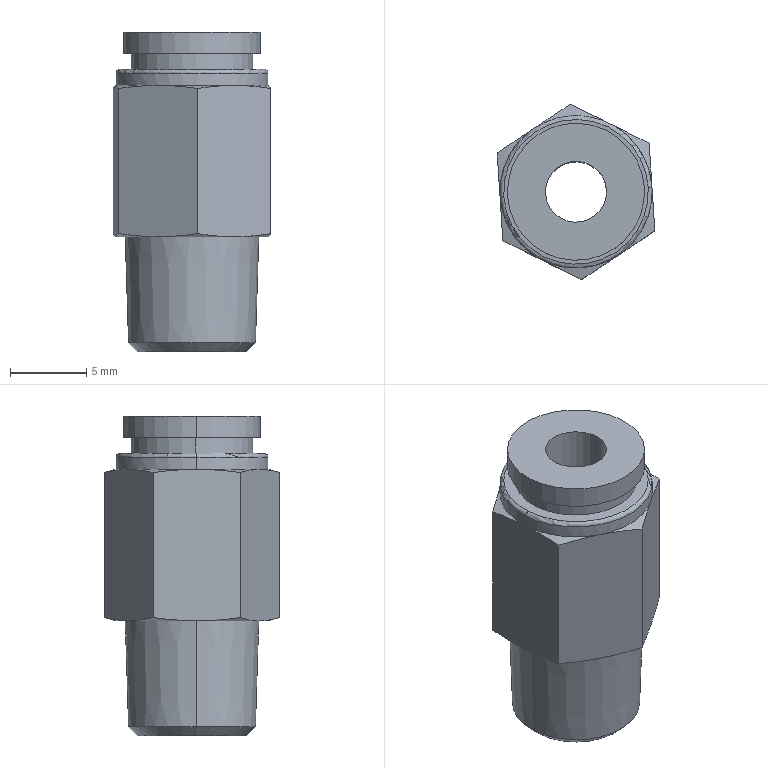Component | SolidWorks | A4-MLCNLSS4-1-L-1 | 1 solid | 37 faces | box 10.35 x 11.52 x 21 mm | volume 1250 mm3 | cone 16 | plane 11 | cylinder 8 | torus 2 | commonest cylinder face diameters 4 x2 9 x2 8 x2 10 x2
STEP:
#1=CARTESIAN_POINT('',(0.07858,-0.3099,2.497));
#2=VERTEX_POINT('',#1);
#3=CARTESIAN_POINT('',(-0.07858,-0.32,2.497));
#4=VERTEX_POINT('',#3);
#5=CARTESIAN_POINT('',(0.,-0.315,2.497));
#6=DIRECTION('',(0.,0.,-1.));
#7=DIRECTION('',(-0.9979,-0.0641,0.));
#8=AXIS2_PLACEMENT_3D('',#5,#6,#7);
#9=CIRCLE('',#8,0.07874);
#10=EDGE_CURVE('',#2,#4,#9,.T.);
#11=ORIENTED_EDGE('',*,*,#10,.F.);
#12=CARTESIAN_POINT('',(0.07858,-0.3099,1.671));
#13=VERTEX_POINT('',#12);
#14=CARTESIAN_POINT('',(0.07858,-0.3099,2.497));
#15=DIRECTION('',(0.,0.,-1.));
#16=VECTOR('',#15,39.37);
#17=LINE('',#14,#16);
#18=EDGE_CURVE('',#2,#13,#17,.T.);
#19=ORIENTED_EDGE('',*,*,#18,.T.);
#20=CARTESIAN_POINT('',(-0.07858,-0.32,1.671));
#21=VERTEX_POINT('',#20);
#22=CARTESIAN_POINT('',(0.,-0.315,1.671));
#23=DIRECTION('',(0.,0.,-1.));
#24=DIRECTION('',(-0.9979,-0.0641,0.));
#25=AXIS2_PLACEMENT_3D('',#22,#23,#24);
#26=CIRCLE('',#25,0.07874);
#27=EDGE_CURVE('',#13,#21,#26,.T.);
#28=ORIENTED_EDGE('',*,*,#27,.T.);
#29=CARTESIAN_POINT('',(-0.07858,-0.32,2.497));
#30=DIRECTION('',(0.,0.,-1.));
#31=VECTOR('',#30,39.37);
#32=LINE('',#29,#31);
#33=EDGE_CURVE('',#4,#21,#32,.T.);
#34=ORIENTED_EDGE('',*,*,#33,.F.);
#35=EDGE_LOOP('',(#11,#19,#28,#34));
#36=FACE_OUTER_BOUND('',#35,.T.);
#37=CARTESIAN_POINT('',(0.,-0.315,2.497));
#38=DIRECTION('',(0.,0.,-1.));
#39=DIRECTION('',(-0.9979,-0.0641,0.));
#40=AXIS2_PLACEMENT_3D('',#37,#38,#39);
#41=CYLINDRICAL_SURFACE('',#40,0.07874);
#42=ADVANCED_FACE('',(#36),#41,.F.);
#43=CARTESIAN_POINT('',(-0.1641,-0.3255,1.694));
#44=VERTEX_POINT('',#43);
#45=CARTESIAN_POINT('',(0.1641,-0.3044,1.694));
#46=VERTEX_POINT('',#45);
#47=CARTESIAN_POINT('',(0.,-0.315,1.694));
#48=DIRECTION('',(0.,0.,-1.));
#49=DIRECTION('',(-0.9979,-0.0641,0.));
#50=AXIS2_PLACEMENT_3D('',#47,#48,#49);
#51=CIRCLE('',#50,0.1644);
#52=EDGE_CURVE('',#44,#46,#51,.T.);
#53=ORIENTED_EDGE('',*,*,#52,.F.);
#54=CARTESIAN_POINT('',(-0.1727,-0.3261,1.969));
#55=VERTEX_POINT('',#54);
#56=CARTESIAN_POINT('',(-0.1727,-0.3261,1.969));
#57=DIRECTION('',(-0.03117,-0.002002,0.9995));
#58=VECTOR('',#57,39.37);
#59=LINE('',#56,#58);
#60=EDGE_CURVE('',#44,#55,#59,.T.);
#61=ORIENTED_EDGE('',*,*,#60,.T.);
#62=CARTESIAN_POINT('',(0.1727,-0.3039,1.969));
#63=VERTEX_POINT('',#62);
#64=CARTESIAN_POINT('',(0.,-0.315,1.969));
#65=DIRECTION('',(0.,0.,-1.));
#66=DIRECTION('',(-0.9979,-0.0641,0.));
#67=AXIS2_PLACEMENT_3D('',#64,#65,#66);
#68=CIRCLE('',#67,0.173);
#69=EDGE_CURVE('',#55,#63,#68,.T.);
#70=ORIENTED_EDGE('',*,*,#69,.T.);
#71=CARTESIAN_POINT('',(0.1727,-0.3039,1.969));
#72=DIRECTION('',(0.03117,0.002002,0.9995));
#73=VECTOR('',#72,39.37);
#74=LINE('',#71,#73);
#75=EDGE_CURVE('',#46,#63,#74,.T.);
#76=ORIENTED_EDGE('',*,*,#75,.F.);
#77=EDGE_LOOP('',(#53,#61,#70,#76));
#78=FACE_OUTER_BOUND('',#77,.T.);
#79=CARTESIAN_POINT('',(0.,-0.315,1.969));
#80=DIRECTION('',(0.,-0.,1.));
#81=DIRECTION('',(0.9979,0.0641,0.));
#82=AXIS2_PLACEMENT_3D('',#79,#80,#81);
#83=CONICAL_SURFACE('',#82,0.173,0.03124);
#84=ADVANCED_FACE('',(#78),#83,.T.);
#85=CARTESIAN_POINT('',(-0.1405,-0.324,1.671));
#86=VERTEX_POINT('',#85);
#87=CARTESIAN_POINT('',(0.1405,-0.3059,1.671));
#88=VERTEX_POINT('',#87);
#89=CARTESIAN_POINT('',(0.,-0.315,1.671));
#90=DIRECTION('',(0.,0.,-1.));
#91=DIRECTION('',(-0.9979,-0.0641,0.));
#92=AXIS2_PLACEMENT_3D('',#89,#90,#91);
#93=CIRCLE('',#92,0.1408);
#94=EDGE_CURVE('',#86,#88,#93,.T.);
#95=ORIENTED_EDGE('',*,*,#94,.F.);
#96=CARTESIAN_POINT('',(-0.1641,-0.3255,1.694));
#97=DIRECTION('',(-0.7057,-0.04533,0.7071));
#98=VECTOR('',#97,39.37);
#99=LINE('',#96,#98);
#100=EDGE_CURVE('',#86,#44,#99,.T.);
#101=ORIENTED_EDGE('',*,*,#100,.T.);
#102=ORIENTED_EDGE('',*,*,#52,.T.);
#103=CARTESIAN_POINT('',(0.1641,-0.3044,1.694));
#104=DIRECTION('',(0.7057,0.04533,0.7071));
#105=VECTOR('',#104,39.37);
#106=LINE('',#103,#105);
#107=EDGE_CURVE('',#88,#46,#106,.T.);
#108=ORIENTED_EDGE('',*,*,#107,.F.);
#109=EDGE_LOOP('',(#95,#101,#102,#108));
#110=FACE_OUTER_BOUND('',#109,.T.);
#111=CARTESIAN_POINT('',(0.,-0.315,1.694));
#112=DIRECTION('',(0.,-0.,1.));
#113=DIRECTION('',(0.9979,0.0641,0.));
#114=AXIS2_PLACEMENT_3D('',#111,#112,#113);
#115=CONICAL_SURFACE('',#114,0.1644,0.7854);
#116=ADVANCED_FACE('',(#110),#115,.T.);
#117=CARTESIAN_POINT('',(-0.1768,-0.3263,2.497));
#118=VERTEX_POINT('',#117);
#119=CARTESIAN_POINT('',(0.1768,-0.3036,2.497));
#120=VERTEX_POINT('',#119);
#121=CARTESIAN_POINT('',(0.,-0.315,2.497));
#122=DIRECTION('',(0.,0.,-1.));
#123=DIRECTION('',(-0.9979,-0.0641,0.));
#124=AXIS2_PLACEMENT_3D('',#121,#122,#123);
#125=CIRCLE('',#124,0.1772);
#126=EDGE_CURVE('',#118,#120,#125,.T.);
#127=ORIENTED_EDGE('',*,*,#126,.T.);
#128=CARTESIAN_POINT('',(0.1768,-0.3036,2.442));
#129=VERTEX_POINT('',#128);
#130=CARTESIAN_POINT('',(0.1768,-0.3036,2.497));
#131=DIRECTION('',(0.,0.,-1.));
#132=VECTOR('',#131,39.37);
#133=LINE('',#130,#132);
#134=EDGE_CURVE('',#120,#129,#133,.T.);
#135=ORIENTED_EDGE('',*,*,#134,.T.);
#136=CARTESIAN_POINT('',(-0.1768,-0.3263,2.442));
#137=VERTEX_POINT('',#136);
#138=CARTESIAN_POINT('',(0.,-0.315,2.442));
#139=DIRECTION('',(0.,0.,-1.));
#140=DIRECTION('',(-0.9979,-0.0641,0.));
#141=AXIS2_PLACEMENT_3D('',#138,#139,#140);
#142=CIRCLE('',#141,0.1772);
#143=EDGE_CURVE('',#137,#129,#142,.T.);
#144=ORIENTED_EDGE('',*,*,#143,.F.);
#145=CARTESIAN_POINT('',(-0.1768,-0.3263,2.497));
#146=DIRECTION('',(0.,0.,-1.));
#147=VECTOR('',#146,39.37);
#148=LINE('',#145,#147);
#149=EDGE_CURVE('',#118,#137,#148,.T.);
#150=ORIENTED_EDGE('',*,*,#149,.F.);
#151=EDGE_LOOP('',(#127,#135,#144,#150));
#152=FACE_OUTER_BOUND('',#151,.T.);
#153=CARTESIAN_POINT('',(0.,-0.315,2.497));
#154=DIRECTION('',(0.,0.,-1.));
#155=DIRECTION('',(-0.9979,-0.0641,0.));
#156=AXIS2_PLACEMENT_3D('',#153,#154,#155);
#157=CYLINDRICAL_SURFACE('',#156,0.1772);
#158=ADVANCED_FACE('',(#152),#157,.T.);
#159=CARTESIAN_POINT('',(-0.1572,-0.3251,2.442));
#160=VERTEX_POINT('',#159);
#161=CARTESIAN_POINT('',(0.1572,-0.3049,2.442));
#162=VERTEX_POINT('',#161);
#163=CARTESIAN_POINT('',(0.,-0.315,2.442));
#164=DIRECTION('',(0.,0.,-1.));
#165=DIRECTION('',(-0.9979,-0.0641,0.));
#166=AXIS2_PLACEMENT_3D('',#163,#164,#165);
#167=CIRCLE('',#166,0.1575);
#168=EDGE_CURVE('',#160,#162,#167,.T.);
#169=ORIENTED_EDGE('',*,*,#168,.T.);
#170=CARTESIAN_POINT('',(0.1572,-0.3049,2.401));
#171=VERTEX_POINT('',#170);
#172=CARTESIAN_POINT('',(0.1572,-0.3049,2.497));
#173=DIRECTION('',(0.,0.,-1.));
#174=VECTOR('',#173,39.37);
#175=LINE('',#172,#174);
#176=EDGE_CURVE('',#162,#171,#175,.T.);
#177=ORIENTED_EDGE('',*,*,#176,.T.);
#178=CARTESIAN_POINT('',(-0.1572,-0.3251,2.401));
#179=VERTEX_POINT('',#178);
#180=CARTESIAN_POINT('',(0.,-0.315,2.401));
#181=DIRECTION('',(0.,0.,-1.));
#182=DIRECTION('',(-0.9979,-0.0641,0.));
#183=AXIS2_PLACEMENT_3D('',#180,#181,#182);
#184=CIRCLE('',#183,0.1575);
#185=EDGE_CURVE('',#179,#171,#184,.T.);
#186=ORIENTED_EDGE('',*,*,#185,.F.);
#187=CARTESIAN_POINT('',(-0.1572,-0.3251,2.497));
#188=DIRECTION('',(0.,0.,-1.));
#189=VECTOR('',#188,39.37);
#190=LINE('',#187,#189);
#191=EDGE_CURVE('',#160,#179,#190,.T.);
#192=ORIENTED_EDGE('',*,*,#191,.F.);
#193=EDGE_LOOP('',(#169,#177,#186,#192));
#194=FACE_OUTER_BOUND('',#193,.T.);
#195=CARTESIAN_POINT('',(0.,-0.315,2.497));
#196=DIRECTION('',(0.,0.,-1.));
#197=DIRECTION('',(-0.9979,-0.0641,0.));
#198=AXIS2_PLACEMENT_3D('',#195,#196,#197);
#199=CYLINDRICAL_SURFACE('',#198,0.1575);
#200=ADVANCED_FACE('',(#194),#199,.T.);
#201=CARTESIAN_POINT('',(-0.1866,-0.3269,2.401));
#202=VERTEX_POINT('',#201);
#203=CARTESIAN_POINT('',(0.1866,-0.303,2.401));
#204=VERTEX_POINT('',#203);
#205=CARTESIAN_POINT('',(0.,-0.315,2.401));
#206=DIRECTION('',(0.,0.,-1.));
#207=DIRECTION('',(-0.9979,-0.0641,0.));
#208=AXIS2_PLACEMENT_3D('',#205,#206,#207);
#209=CIRCLE('',#208,0.187);
#210=EDGE_CURVE('',#202,#204,#209,.T.);
#211=ORIENTED_EDGE('',*,*,#210,.T.);
#212=CARTESIAN_POINT('',(0.1964,-0.3023,2.391));
#213=VERTEX_POINT('',#212);
#214=CARTESIAN_POINT('',(0.1866,-0.303,2.391));
#215=DIRECTION('',(-0.0641,0.9979,0.));
#216=DIRECTION('',(-0.9979,-0.0641,0.));
#217=AXIS2_PLACEMENT_3D('',#214,#215,#216);
#218=CIRCLE('',#217,0.009843);
#219=EDGE_CURVE('',#204,#213,#218,.T.);
#220=ORIENTED_EDGE('',*,*,#219,.T.);
#221=CARTESIAN_POINT('',(-0.1964,-0.3276,2.391));
#222=VERTEX_POINT('',#221);
#223=CARTESIAN_POINT('',(0.,-0.315,2.391));
#224=DIRECTION('',(0.,0.,-1.));
#225=DIRECTION('',(-0.9979,-0.0641,0.));
#226=AXIS2_PLACEMENT_3D('',#223,#224,#225);
#227=CIRCLE('',#226,0.1969);
#228=EDGE_CURVE('',#222,#213,#227,.T.);
#229=ORIENTED_EDGE('',*,*,#228,.F.);
#230=CARTESIAN_POINT('',(-0.1866,-0.3269,2.391));
#231=DIRECTION('',(0.0641,-0.9979,-0.));
#232=DIRECTION('',(0.9979,0.0641,0.));
#233=AXIS2_PLACEMENT_3D('',#230,#231,#232);
#234=CIRCLE('',#233,0.009843);
#235=EDGE_CURVE('',#202,#222,#234,.T.);
#236=ORIENTED_EDGE('',*,*,#235,.F.);
#237=EDGE_LOOP('',(#211,#220,#229,#236));
#238=FACE_OUTER_BOUND('',#237,.T.);
#239=CARTESIAN_POINT('',(0.,-0.315,2.391));
#240=DIRECTION('',(0.,0.,-1.));
#241=DIRECTION('',(-0.9979,-0.0641,-0.));
#242=AXIS2_PLACEMENT_3D('',#239,#240,#241);
#243=TOROIDAL_SURFACE('',#242,0.187,0.009843);
#244=ADVANCED_FACE('',(#238),#243,.T.);
#245=ORIENTED_EDGE('',*,*,#228,.T.);
#246=CARTESIAN_POINT('',(0.1964,-0.3023,2.36));
#247=VERTEX_POINT('',#246);
#248=CARTESIAN_POINT('',(0.1964,-0.3023,2.497));
#249=DIRECTION('',(0.,0.,-1.));
#250=VECTOR('',#249,39.37);
#251=LINE('',#248,#250);
#252=EDGE_CURVE('',#213,#247,#251,.T.);
#253=ORIENTED_EDGE('',*,*,#252,.T.);
#254=CARTESIAN_POINT('',(0.08729,-0.1385,2.36));
#255=VERTEX_POINT('',#254);
#256=CARTESIAN_POINT('',(0.,-0.315,2.36));
#257=DIRECTION('',(0.,0.,-1.));
#258=DIRECTION('',(-0.9979,-0.0641,0.));
#259=AXIS2_PLACEMENT_3D('',#256,#257,#258);
#260=CIRCLE('',#259,0.1969);
#261=EDGE_CURVE('',#255,#247,#260,.T.);
#262=ORIENTED_EDGE('',*,*,#261,.F.);
#263=CARTESIAN_POINT('',(-0.1092,-0.1511,2.36));
#264=VERTEX_POINT('',#263);
#265=CARTESIAN_POINT('',(0.,-0.315,2.36));
#266=DIRECTION('',(0.,0.,-1.));
#267=DIRECTION('',(-0.9979,-0.0641,0.));
#268=AXIS2_PLACEMENT_3D('',#265,#266,#267);
#269=CIRCLE('',#268,0.1969);
#270=EDGE_CURVE('',#264,#255,#269,.T.);
#271=ORIENTED_EDGE('',*,*,#270,.F.);
#272=CARTESIAN_POINT('',(-0.1964,-0.3276,2.36));
#273=VERTEX_POINT('',#272);
#274=CARTESIAN_POINT('',(0.,-0.315,2.36));
#275=DIRECTION('',(0.,0.,-1.));
#276=DIRECTION('',(-0.9979,-0.0641,0.));
#277=AXIS2_PLACEMENT_3D('',#274,#275,#276);
#278=CIRCLE('',#277,0.1969);
#279=EDGE_CURVE('',#273,#264,#278,.T.);
#280=ORIENTED_EDGE('',*,*,#279,.F.);
#281=CARTESIAN_POINT('',(-0.1964,-0.3276,2.497));
#282=DIRECTION('',(0.,0.,-1.));
#283=VECTOR('',#282,39.37);
#284=LINE('',#281,#283);
#285=EDGE_CURVE('',#222,#273,#284,.T.);
#286=ORIENTED_EDGE('',*,*,#285,.F.);
#287=EDGE_LOOP('',(#245,#253,#262,#271,#280,#286));
#288=FACE_OUTER_BOUND('',#287,.T.);
#289=CARTESIAN_POINT('',(0.,-0.315,2.497));
#290=DIRECTION('',(0.,0.,-1.));
#291=DIRECTION('',(-0.9979,-0.0641,0.));
#292=AXIS2_PLACEMENT_3D('',#289,#290,#291);
#293=CYLINDRICAL_SURFACE('',#292,0.1969);
#294=ADVANCED_FACE('',(#288),#293,.T.);
#295=ORIENTED_EDGE('',*,*,#126,.F.);
#296=CARTESIAN_POINT('',(0.,-0.315,2.497));
#297=DIRECTION('',(0.,0.,-1.));
#298=DIRECTION('',(-0.9979,-0.0641,0.));
#299=AXIS2_PLACEMENT_3D('',#296,#297,#298);
#300=CIRCLE('',#299,0.1772);
#301=EDGE_CURVE('',#120,#118,#300,.T.);
#302=ORIENTED_EDGE('',*,*,#301,.F.);
#303=EDGE_LOOP('',(#295,#302));
#304=FACE_OUTER_BOUND('',#303,.T.);
#305=CARTESIAN_POINT('',(0.,-0.315,2.497));
#306=DIRECTION('',(0.,0.,-1.));
#307=DIRECTION('',(-0.9979,-0.0641,0.));
#308=AXIS2_PLACEMENT_3D('',#305,#306,#307);
#309=CIRCLE('',#308,0.07874);
#310=EDGE_CURVE('',#4,#2,#309,.T.);
#311=ORIENTED_EDGE('',*,*,#310,.T.);
#312=ORIENTED_EDGE('',*,*,#10,.T.);
#313=EDGE_LOOP('',(#311,#312));
#314=FACE_BOUND('',#313,.T.);
#315=CARTESIAN_POINT('',(-0.01136,-0.1382,2.497));
#316=DIRECTION('',(0.,0.,-1.));
#317=DIRECTION('',(-0.9979,-0.0641,-0.));
#318=AXIS2_PLACEMENT_3D('',#315,#316,#317);
#319=PLANE('',#318);
#320=ADVANCED_FACE('',(#304,#314),#319,.F.);
#321=CARTESIAN_POINT('',(0.,-0.315,1.671));
#322=DIRECTION('',(0.,0.,-1.));
#323=DIRECTION('',(-0.9979,-0.0641,0.));
#324=AXIS2_PLACEMENT_3D('',#321,#322,#323);
#325=CIRCLE('',#324,0.1408);
#326=EDGE_CURVE('',#88,#86,#325,.T.);
#327=ORIENTED_EDGE('',*,*,#326,.T.);
#328=ORIENTED_EDGE('',*,*,#94,.T.);
#329=EDGE_LOOP('',(#327,#328));
#330=FACE_OUTER_BOUND('',#329,.T.);
#331=CARTESIAN_POINT('',(0.,-0.315,1.671));
#332=DIRECTION('',(0.,0.,-1.));
#333=DIRECTION('',(-0.9979,-0.0641,0.));
#334=AXIS2_PLACEMENT_3D('',#331,#332,#333);
#335=CIRCLE('',#334,0.07874);
#336=EDGE_CURVE('',#21,#13,#335,.T.);
#337=ORIENTED_EDGE('',*,*,#336,.F.);
#338=ORIENTED_EDGE('',*,*,#27,.F.);
#339=EDGE_LOOP('',(#337,#338));
#340=FACE_BOUND('',#339,.T.);
#341=CARTESIAN_POINT('',(0.,-0.315,1.671));
#342=DIRECTION('',(-0.,-0.,1.));
#343=DIRECTION('',(0.9979,0.0641,0.));
#344=AXIS2_PLACEMENT_3D('',#341,#342,#343);
#345=PLANE('',#344);
#346=ADVANCED_FACE('',(#330,#340),#345,.F.);
#347=CARTESIAN_POINT('',(-0.2037,-0.2142,2.352));
#348=VERTEX_POINT('',#347);
#349=CARTESIAN_POINT('',(-0.2037,-0.2142,2.352));
#350=CARTESIAN_POINT('',(-0.1722,-0.1932,2.357));
#351=CARTESIAN_POINT('',(-0.1407,-0.1721,2.36));
#352=CARTESIAN_POINT('',(-0.1092,-0.1511,2.36));
#353=B_SPLINE_CURVE_WITH_KNOTS('',3,(#349,#350,#351,#352),.UNSPECIFIED.,.F.,.F.,(4,4),(0.00000023,0.002887),.UNSPECIFIED.);
#354=EDGE_CURVE('',#348,#264,#353,.T.);
#355=ORIENTED_EDGE('',*,*,#354,.F.);
#356=CARTESIAN_POINT('',(-0.1964,-0.3276,2.36));
#357=CARTESIAN_POINT('',(-0.1989,-0.2897,2.36));
#358=CARTESIAN_POINT('',(-0.2013,-0.2519,2.357));
#359=CARTESIAN_POINT('',(-0.2037,-0.2142,2.352));
#360=B_SPLINE_CURVE_WITH_KNOTS('',3,(#356,#357,#358,#359),.UNSPECIFIED.,.F.,.F.,(4,4),(0.007734,0.01065),.UNSPECIFIED.);
#361=EDGE_CURVE('',#273,#348,#360,.T.);
#362=ORIENTED_EDGE('',*,*,#361,.F.);
#363=ORIENTED_EDGE('',*,*,#279,.T.);
#364=EDGE_LOOP('',(#355,#362,#363));
#365=FACE_OUTER_BOUND('',#364,.T.);
#366=CARTESIAN_POINT('',(0.,-0.315,2.36));
#367=DIRECTION('',(0.,0.,-1.));
#368=DIRECTION('',(-0.9979,-0.0641,0.));
#369=AXIS2_PLACEMENT_3D('',#366,#367,#368);
#370=CONICAL_SURFACE('',#369,0.1969,1.309);
#371=ADVANCED_FACE('',(#365),#370,.T.);
#372=CARTESIAN_POINT('',(-0.01457,-0.08812,2.352));
#373=VERTEX_POINT('',#372);
#374=CARTESIAN_POINT('',(-0.1092,-0.1511,2.36));
#375=CARTESIAN_POINT('',(-0.07762,-0.1301,2.36));
#376=CARTESIAN_POINT('',(-0.0461,-0.1091,2.357));
#377=CARTESIAN_POINT('',(-0.01457,-0.08812,2.352));
#378=B_SPLINE_CURVE_WITH_KNOTS('',3,(#374,#375,#376,#377),.UNSPECIFIED.,.F.,.F.,(4,4),(0.002887,0.005774),.UNSPECIFIED.);
#379=EDGE_CURVE('',#264,#373,#378,.T.);
#380=ORIENTED_EDGE('',*,*,#379,.F.);
#381=ORIENTED_EDGE('',*,*,#270,.T.);
#382=CARTESIAN_POINT('',(-0.01457,-0.08812,2.352));
#383=CARTESIAN_POINT('',(0.01938,-0.1049,2.357));
#384=CARTESIAN_POINT('',(0.05334,-0.1217,2.36));
#385=CARTESIAN_POINT('',(0.08729,-0.1385,2.36));
#386=B_SPLINE_CURVE_WITH_KNOTS('',3,(#382,#383,#384,#385),.UNSPECIFIED.,.F.,.F.,(4,4),(0.00000023,0.002887),.UNSPECIFIED.);
#387=EDGE_CURVE('',#373,#255,#386,.T.);
#388=ORIENTED_EDGE('',*,*,#387,.F.);
#389=EDGE_LOOP('',(#380,#381,#388));
#390=FACE_OUTER_BOUND('',#389,.T.);
#391=CARTESIAN_POINT('',(0.,-0.315,2.36));
#392=DIRECTION('',(0.,0.,-1.));
#393=DIRECTION('',(-0.9979,-0.0641,0.));
#394=AXIS2_PLACEMENT_3D('',#391,#392,#393);
#395=CONICAL_SURFACE('',#394,0.1969,1.309);
#396=ADVANCED_FACE('',(#390),#395,.T.);
#397=CARTESIAN_POINT('',(0.1892,-0.1889,2.352));
#398=VERTEX_POINT('',#397);
#399=CARTESIAN_POINT('',(0.08729,-0.1385,2.36));
#400=CARTESIAN_POINT('',(0.1213,-0.1553,2.36));
#401=CARTESIAN_POINT('',(0.1552,-0.1721,2.357));
#402=CARTESIAN_POINT('',(0.1892,-0.1889,2.352));
#403=B_SPLINE_CURVE_WITH_KNOTS('',3,(#399,#400,#401,#402),.UNSPECIFIED.,.F.,.F.,(4,4),(0.002887,0.005774),.UNSPECIFIED.);
#404=EDGE_CURVE('',#255,#398,#403,.T.);
#405=ORIENTED_EDGE('',*,*,#404,.F.);
#406=ORIENTED_EDGE('',*,*,#261,.T.);
#407=CARTESIAN_POINT('',(0.1892,-0.1889,2.352));
#408=CARTESIAN_POINT('',(0.1916,-0.2267,2.357));
#409=CARTESIAN_POINT('',(0.194,-0.2645,2.36));
#410=CARTESIAN_POINT('',(0.1964,-0.3023,2.36));
#411=B_SPLINE_CURVE_WITH_KNOTS('',3,(#407,#408,#409,#410),.UNSPECIFIED.,.F.,.F.,(4,4),(0.01099,0.0139),.UNSPECIFIED.);
#412=EDGE_CURVE('',#398,#247,#411,.T.);
#413=ORIENTED_EDGE('',*,*,#412,.F.);
#414=EDGE_LOOP('',(#405,#406,#413));
#415=FACE_OUTER_BOUND('',#414,.T.);
#416=CARTESIAN_POINT('',(0.,-0.315,2.36));
#417=DIRECTION('',(0.,0.,-1.));
#418=DIRECTION('',(-0.9979,-0.0641,0.));
#419=AXIS2_PLACEMENT_3D('',#416,#417,#418);
#420=CONICAL_SURFACE('',#419,0.1969,1.309);
#421=ADVANCED_FACE('',(#415),#420,.T.);
#422=CARTESIAN_POINT('',(0.2037,-0.4158,2.352));
#423=VERTEX_POINT('',#422);
#424=CARTESIAN_POINT('',(0.1964,-0.3023,2.36));
#425=CARTESIAN_POINT('',(0.1977,-0.3212,2.36));
#426=CARTESIAN_POINT('',(0.1989,-0.3401,2.359));
#427=CARTESIAN_POINT('',(0.2013,-0.378,2.356));
#428=CARTESIAN_POINT('',(0.2025,-0.3969,2.354));
#429=CARTESIAN_POINT('',(0.2037,-0.4158,2.352));
#430=B_SPLINE_CURVE_WITH_KNOTS('',3,(#424,#425,#426,#427,#428,#429),.UNSPECIFIED.,.F.,.F.,(4,2,4),(0.0139,0.01535,0.01679),.UNSPECIFIED.);
#431=EDGE_CURVE('',#247,#423,#430,.T.);
#432=ORIENTED_EDGE('',*,*,#431,.F.);
#433=CARTESIAN_POINT('',(0.1092,-0.4788,2.36));
#434=VERTEX_POINT('',#433);
#435=CARTESIAN_POINT('',(0.,-0.315,2.36));
#436=DIRECTION('',(0.,0.,-1.));
#437=DIRECTION('',(-0.9979,-0.0641,0.));
#438=AXIS2_PLACEMENT_3D('',#435,#436,#437);
#439=CIRCLE('',#438,0.1969);
#440=EDGE_CURVE('',#247,#434,#439,.T.);
#441=ORIENTED_EDGE('',*,*,#440,.T.);
#442=CARTESIAN_POINT('',(0.2037,-0.4158,2.352));
#443=CARTESIAN_POINT('',(0.1722,-0.4368,2.357));
#444=CARTESIAN_POINT('',(0.1407,-0.4578,2.36));
#445=CARTESIAN_POINT('',(0.1092,-0.4788,2.36));
#446=B_SPLINE_CURVE_WITH_KNOTS('',3,(#442,#443,#444,#445),.UNSPECIFIED.,.F.,.F.,(4,4),(0.00000023,0.002887),.UNSPECIFIED.);
#447=EDGE_CURVE('',#423,#434,#446,.T.);
#448=ORIENTED_EDGE('',*,*,#447,.F.);
#449=EDGE_LOOP('',(#432,#441,#448));
#450=FACE_OUTER_BOUND('',#449,.T.);
#451=CARTESIAN_POINT('',(0.,-0.315,2.36));
#452=DIRECTION('',(0.,0.,-1.));
#453=DIRECTION('',(-0.9979,-0.0641,0.));
#454=AXIS2_PLACEMENT_3D('',#451,#452,#453);
#455=CONICAL_SURFACE('',#454,0.1969,1.309);
#456=ADVANCED_FACE('',(#450),#455,.T.);
#457=CARTESIAN_POINT('',(0.01457,-0.5418,2.352));
#458=VERTEX_POINT('',#457);
#459=CARTESIAN_POINT('',(0.1092,-0.4788,2.36));
#460=CARTESIAN_POINT('',(0.07762,-0.4998,2.36));
#461=CARTESIAN_POINT('',(0.0461,-0.5208,2.357));
#462=CARTESIAN_POINT('',(0.01457,-0.5418,2.352));
#463=B_SPLINE_CURVE_WITH_KNOTS('',3,(#459,#460,#461,#462),.UNSPECIFIED.,.F.,.F.,(4,4),(0.002887,0.005774),.UNSPECIFIED.);
#464=EDGE_CURVE('',#434,#458,#463,.T.);
#465=ORIENTED_EDGE('',*,*,#464,.F.);
#466=CARTESIAN_POINT('',(-0.08729,-0.4914,2.36));
#467=VERTEX_POINT('',#466);
#468=CARTESIAN_POINT('',(0.,-0.315,2.36));
#469=DIRECTION('',(0.,0.,-1.));
#470=DIRECTION('',(-0.9979,-0.0641,0.));
#471=AXIS2_PLACEMENT_3D('',#468,#469,#470);
#472=CIRCLE('',#471,0.1969);
#473=EDGE_CURVE('',#434,#467,#472,.T.);
#474=ORIENTED_EDGE('',*,*,#473,.T.);
#475=CARTESIAN_POINT('',(0.01457,-0.5418,2.352));
#476=CARTESIAN_POINT('',(-0.01938,-0.525,2.357));
#477=CARTESIAN_POINT('',(-0.05334,-0.5082,2.36));
#478=CARTESIAN_POINT('',(-0.08729,-0.4914,2.36));
#479=B_SPLINE_CURVE_WITH_KNOTS('',3,(#475,#476,#477,#478),.UNSPECIFIED.,.F.,.F.,(4,4),(0.00000023,0.002887),.UNSPECIFIED.);
#480=EDGE_CURVE('',#458,#467,#479,.T.);
#481=ORIENTED_EDGE('',*,*,#480,.F.);
#482=EDGE_LOOP('',(#465,#474,#481));
#483=FACE_OUTER_BOUND('',#482,.T.);
#484=CARTESIAN_POINT('',(0.,-0.315,2.36));
#485=DIRECTION('',(0.,0.,-1.));
#486=DIRECTION('',(-0.9979,-0.0641,0.));
#487=AXIS2_PLACEMENT_3D('',#484,#485,#486);
#488=CONICAL_SURFACE('',#487,0.1969,1.309);
#489=ADVANCED_FACE('',(#483),#488,.T.);
#490=CARTESIAN_POINT('',(-0.1892,-0.441,2.352));
#491=VERTEX_POINT('',#490);
#492=CARTESIAN_POINT('',(-0.08729,-0.4914,2.36));
#493=CARTESIAN_POINT('',(-0.1213,-0.4746,2.36));
#494=CARTESIAN_POINT('',(-0.1552,-0.4578,2.357));
#495=CARTESIAN_POINT('',(-0.1892,-0.441,2.352));
#496=B_SPLINE_CURVE_WITH_KNOTS('',3,(#492,#493,#494,#495),.UNSPECIFIED.,.F.,.F.,(4,4),(0.002887,0.005774),.UNSPECIFIED.);
#497=EDGE_CURVE('',#467,#491,#496,.T.);
#498=ORIENTED_EDGE('',*,*,#497,.F.);
#499=CARTESIAN_POINT('',(0.,-0.315,2.36));
#500=DIRECTION('',(0.,0.,-1.));
#501=DIRECTION('',(-0.9979,-0.0641,0.));
#502=AXIS2_PLACEMENT_3D('',#499,#500,#501);
#503=CIRCLE('',#502,0.1969);
#504=EDGE_CURVE('',#467,#273,#503,.T.);
#505=ORIENTED_EDGE('',*,*,#504,.T.);
#506=CARTESIAN_POINT('',(-0.1892,-0.441,2.352));
#507=CARTESIAN_POINT('',(-0.1904,-0.4222,2.354));
#508=CARTESIAN_POINT('',(-0.1916,-0.4032,2.356));
#509=CARTESIAN_POINT('',(-0.194,-0.3654,2.359));
#510=CARTESIAN_POINT('',(-0.1952,-0.3465,2.36));
#511=CARTESIAN_POINT('',(-0.1964,-0.3276,2.36));
#512=B_SPLINE_CURVE_WITH_KNOTS('',3,(#506,#507,#508,#509,#510,#511),.UNSPECIFIED.,.F.,.F.,(4,2,4),(0.004834,0.006284,0.007734),.UNSPECIFIED.);
#513=EDGE_CURVE('',#491,#273,#512,.T.);
#514=ORIENTED_EDGE('',*,*,#513,.F.);
#515=EDGE_LOOP('',(#498,#505,#514));
#516=FACE_OUTER_BOUND('',#515,.T.);
#517=CARTESIAN_POINT('',(0.,-0.315,2.36));
#518=DIRECTION('',(0.,0.,-1.));
#519=DIRECTION('',(-0.9979,-0.0641,0.));
#520=AXIS2_PLACEMENT_3D('',#517,#518,#519);
#521=CONICAL_SURFACE('',#520,0.1969,1.309);
#522=ADVANCED_FACE('',(#516),#521,.T.);
#523=ORIENTED_EDGE('',*,*,#252,.F.);
#524=CARTESIAN_POINT('',(0.,-0.315,2.391));
#525=DIRECTION('',(0.,0.,-1.));
#526=DIRECTION('',(-0.9979,-0.0641,0.));
#527=AXIS2_PLACEMENT_3D('',#524,#525,#526);
#528=CIRCLE('',#527,0.1969);
#529=EDGE_CURVE('',#213,#222,#528,.T.);
#530=ORIENTED_EDGE('',*,*,#529,.T.);
#531=ORIENTED_EDGE('',*,*,#285,.T.);
#532=ORIENTED_EDGE('',*,*,#504,.F.);
#533=ORIENTED_EDGE('',*,*,#473,.F.);
#534=ORIENTED_EDGE('',*,*,#440,.F.);
#535=EDGE_LOOP('',(#523,#530,#531,#532,#533,#534));
#536=FACE_OUTER_BOUND('',#535,.T.);
#537=CARTESIAN_POINT('',(0.,-0.315,2.497));
#538=DIRECTION('',(0.,0.,-1.));
#539=DIRECTION('',(-0.9979,-0.0641,0.));
#540=AXIS2_PLACEMENT_3D('',#537,#538,#539);
#541=CYLINDRICAL_SURFACE('',#540,0.1969);
#542=ADVANCED_FACE('',(#536),#541,.T.);
#543=ORIENTED_EDGE('',*,*,#219,.F.);
#544=CARTESIAN_POINT('',(0.,-0.315,2.401));
#545=DIRECTION('',(0.,0.,-1.));
#546=DIRECTION('',(-0.9979,-0.0641,0.));
#547=AXIS2_PLACEMENT_3D('',#544,#545,#546);
#548=CIRCLE('',#547,0.187);
#549=EDGE_CURVE('',#204,#202,#548,.T.);
#550=ORIENTED_EDGE('',*,*,#549,.T.);
#551=ORIENTED_EDGE('',*,*,#235,.T.);
#552=ORIENTED_EDGE('',*,*,#529,.F.);
#553=EDGE_LOOP('',(#543,#550,#551,#552));
#554=FACE_OUTER_BOUND('',#553,.T.);
#555=CARTESIAN_POINT('',(0.,-0.315,2.391));
#556=DIRECTION('',(0.,0.,-1.));
#557=DIRECTION('',(-0.9979,-0.0641,-0.));
#558=AXIS2_PLACEMENT_3D('',#555,#556,#557);
#559=TOROIDAL_SURFACE('',#558,0.187,0.009843);
#560=ADVANCED_FACE('',(#554),#559,.T.);
#561=ORIENTED_EDGE('',*,*,#210,.F.);
#562=ORIENTED_EDGE('',*,*,#549,.F.);
#563=EDGE_LOOP('',(#561,#562));
#564=FACE_OUTER_BOUND('',#563,.T.);
#565=ORIENTED_EDGE('',*,*,#185,.T.);
#566=CARTESIAN_POINT('',(0.,-0.315,2.401));
#567=DIRECTION('',(0.,0.,-1.));
#568=DIRECTION('',(-0.9979,-0.0641,0.));
#569=AXIS2_PLACEMENT_3D('',#566,#567,#568);
#570=CIRCLE('',#569,0.1575);
#571=EDGE_CURVE('',#171,#179,#570,.T.);
#572=ORIENTED_EDGE('',*,*,#571,.T.);
#573=EDGE_LOOP('',(#565,#572));
#574=FACE_BOUND('',#573,.T.);
#575=CARTESIAN_POINT('',(-0.01199,-0.1283,2.401));
#576=DIRECTION('',(0.,0.,-1.));
#577=DIRECTION('',(-0.9979,-0.0641,-0.));
#578=AXIS2_PLACEMENT_3D('',#575,#576,#577);
#579=PLANE('',#578);
#580=ADVANCED_FACE('',(#564,#574),#579,.F.);
#581=ORIENTED_EDGE('',*,*,#176,.F.);
#582=CARTESIAN_POINT('',(0.,-0.315,2.442));
#583=DIRECTION('',(0.,0.,-1.));
#584=DIRECTION('',(-0.9979,-0.0641,0.));
#585=AXIS2_PLACEMENT_3D('',#582,#583,#584);
#586=CIRCLE('',#585,0.1575);
#587=EDGE_CURVE('',#162,#160,#586,.T.);
#588=ORIENTED_EDGE('',*,*,#587,.T.);
#589=ORIENTED_EDGE('',*,*,#191,.T.);
#590=ORIENTED_EDGE('',*,*,#571,.F.);
#591=EDGE_LOOP('',(#581,#588,#589,#590));
#592=FACE_OUTER_BOUND('',#591,.T.);
#593=CARTESIAN_POINT('',(0.,-0.315,2.497));
#594=DIRECTION('',(0.,0.,-1.));
#595=DIRECTION('',(-0.9979,-0.0641,0.));
#596=AXIS2_PLACEMENT_3D('',#593,#594,#595);
#597=CYLINDRICAL_SURFACE('',#596,0.1575);
#598=ADVANCED_FACE('',(#592),#597,.T.);
#599=ORIENTED_EDGE('',*,*,#168,.F.);
#600=ORIENTED_EDGE('',*,*,#587,.F.);
#601=EDGE_LOOP('',(#599,#600));
#602=FACE_BOUND('',#601,.T.);
#603=ORIENTED_EDGE('',*,*,#143,.T.);
#604=CARTESIAN_POINT('',(0.,-0.315,2.442));
#605=DIRECTION('',(0.,0.,-1.));
#606=DIRECTION('',(-0.9979,-0.0641,0.));
#607=AXIS2_PLACEMENT_3D('',#604,#605,#606);
#608=CIRCLE('',#607,0.1772);
#609=EDGE_CURVE('',#129,#137,#608,.T.);
#610=ORIENTED_EDGE('',*,*,#609,.T.);
#611=EDGE_LOOP('',(#603,#610));
#612=FACE_OUTER_BOUND('',#611,.T.);
#613=CARTESIAN_POINT('',(-0.01009,-0.1578,2.442));
#614=DIRECTION('',(-0.,-0.,1.));
#615=DIRECTION('',(0.9979,0.0641,0.));
#616=AXIS2_PLACEMENT_3D('',#613,#614,#615);
#617=PLANE('',#616);
#618=ADVANCED_FACE('',(#602,#612),#617,.F.);
#619=ORIENTED_EDGE('',*,*,#134,.F.);
#620=ORIENTED_EDGE('',*,*,#301,.T.);
#621=ORIENTED_EDGE('',*,*,#149,.T.);
#622=ORIENTED_EDGE('',*,*,#609,.F.);
#623=EDGE_LOOP('',(#619,#620,#621,#622));
#624=FACE_OUTER_BOUND('',#623,.T.);
#625=CARTESIAN_POINT('',(0.,-0.315,2.497));
#626=DIRECTION('',(0.,0.,-1.));
#627=DIRECTION('',(-0.9979,-0.0641,0.));
#628=AXIS2_PLACEMENT_3D('',#625,#626,#627);
#629=CYLINDRICAL_SURFACE('',#628,0.1772);
#630=ADVANCED_FACE('',(#624),#629,.T.);
#631=CARTESIAN_POINT('',(-0.01457,-0.08812,1.977));
#632=VERTEX_POINT('',#631);
#633=CARTESIAN_POINT('',(-0.1092,-0.1511,1.969));
#634=VERTEX_POINT('',#633);
#635=CARTESIAN_POINT('',(-0.01457,-0.08812,1.977));
#636=CARTESIAN_POINT('',(-0.0461,-0.1091,1.972));
#637=CARTESIAN_POINT('',(-0.07762,-0.1301,1.969));
#638=CARTESIAN_POINT('',(-0.1092,-0.1511,1.969));
#639=B_SPLINE_CURVE_WITH_KNOTS('',3,(#635,#636,#637,#638),.UNSPECIFIED.,.F.,.F.,(4,4),(0.00000023,0.002887),.UNSPECIFIED.);
#640=EDGE_CURVE('',#632,#634,#639,.T.);
#641=ORIENTED_EDGE('',*,*,#640,.T.);
#642=CARTESIAN_POINT('',(-0.2037,-0.2142,1.977));
#643=VERTEX_POINT('',#642);
#644=CARTESIAN_POINT('',(-0.1092,-0.1511,1.969));
#645=CARTESIAN_POINT('',(-0.1407,-0.1721,1.969));
#646=CARTESIAN_POINT('',(-0.1722,-0.1932,1.972));
#647=CARTESIAN_POINT('',(-0.2037,-0.2142,1.977));
#648=B_SPLINE_CURVE_WITH_KNOTS('',3,(#644,#645,#646,#647),.UNSPECIFIED.,.F.,.F.,(4,4),(0.002887,0.005774),.UNSPECIFIED.);
#649=EDGE_CURVE('',#634,#643,#648,.T.);
#650=ORIENTED_EDGE('',*,*,#649,.T.);
#651=CARTESIAN_POINT('',(-0.2037,-0.2142,1.809));
#652=DIRECTION('',(0.,-0.,1.));
#653=VECTOR('',#652,39.37);
#654=LINE('',#651,#653);
#655=EDGE_CURVE('',#643,#348,#654,.T.);
#656=ORIENTED_EDGE('',*,*,#655,.T.);
#657=ORIENTED_EDGE('',*,*,#354,.T.);
#658=ORIENTED_EDGE('',*,*,#379,.T.);
#659=CARTESIAN_POINT('',(-0.01457,-0.08812,1.809));
#660=DIRECTION('',(0.,-0.,1.));
#661=VECTOR('',#660,39.37);
#662=LINE('',#659,#661);
#663=EDGE_CURVE('',#632,#373,#662,.T.);
#664=ORIENTED_EDGE('',*,*,#663,.F.);
#665=EDGE_LOOP('',(#641,#650,#656,#657,#658,#664));
#666=FACE_OUTER_BOUND('',#665,.T.);
#667=CARTESIAN_POINT('',(-0.01457,-0.08812,1.809));
#668=DIRECTION('',(-0.5545,0.8322,0.));
#669=DIRECTION('',(-0.8322,-0.5545,-0.));
#670=AXIS2_PLACEMENT_3D('',#667,#668,#669);
#671=PLANE('',#670);
#672=ADVANCED_FACE('',(#666),#671,.T.);
#673=CARTESIAN_POINT('',(0.1892,-0.1889,1.977));
#674=VERTEX_POINT('',#673);
#675=CARTESIAN_POINT('',(0.08729,-0.1385,1.969));
#676=VERTEX_POINT('',#675);
#677=CARTESIAN_POINT('',(0.1892,-0.1889,1.977));
#678=CARTESIAN_POINT('',(0.1552,-0.1721,1.972));
#679=CARTESIAN_POINT('',(0.1213,-0.1553,1.969));
#680=CARTESIAN_POINT('',(0.08729,-0.1385,1.969));
#681=B_SPLINE_CURVE_WITH_KNOTS('',3,(#677,#678,#679,#680),.UNSPECIFIED.,.F.,.F.,(4,4),(0.00000023,0.002887),.UNSPECIFIED.);
#682=EDGE_CURVE('',#674,#676,#681,.T.);
#683=ORIENTED_EDGE('',*,*,#682,.T.);
#684=CARTESIAN_POINT('',(0.08729,-0.1385,1.969));
#685=CARTESIAN_POINT('',(0.05334,-0.1217,1.969));
#686=CARTESIAN_POINT('',(0.01938,-0.1049,1.972));
#687=CARTESIAN_POINT('',(-0.01457,-0.08812,1.977));
#688=B_SPLINE_CURVE_WITH_KNOTS('',3,(#684,#685,#686,#687),.UNSPECIFIED.,.F.,.F.,(4,4),(0.002887,0.005774),.UNSPECIFIED.);
#689=EDGE_CURVE('',#676,#632,#688,.T.);
#690=ORIENTED_EDGE('',*,*,#689,.T.);
#691=ORIENTED_EDGE('',*,*,#663,.T.);
#692=ORIENTED_EDGE('',*,*,#387,.T.);
#693=ORIENTED_EDGE('',*,*,#404,.T.);
#694=CARTESIAN_POINT('',(0.1892,-0.1889,1.809));
#695=DIRECTION('',(0.,-0.,1.));
#696=VECTOR('',#695,39.37);
#697=LINE('',#694,#696);
#698=EDGE_CURVE('',#674,#398,#697,.T.);
#699=ORIENTED_EDGE('',*,*,#698,.F.);
#700=EDGE_LOOP('',(#683,#690,#691,#692,#693,#699));
#701=FACE_OUTER_BOUND('',#700,.T.);
#702=CARTESIAN_POINT('',(0.1892,-0.1889,1.809));
#703=DIRECTION('',(0.4435,0.8963,0.));
#704=DIRECTION('',(-0.8963,0.4435,0.));
#705=AXIS2_PLACEMENT_3D('',#702,#703,#704);
#706=PLANE('',#705);
#707=ADVANCED_FACE('',(#701),#706,.T.);
#708=CARTESIAN_POINT('',(0.2037,-0.4158,1.977));
#709=VERTEX_POINT('',#708);
#710=CARTESIAN_POINT('',(0.1964,-0.3023,1.969));
#711=VERTEX_POINT('',#710);
#712=CARTESIAN_POINT('',(0.2037,-0.4158,1.977));
#713=CARTESIAN_POINT('',(0.2025,-0.3969,1.974));
#714=CARTESIAN_POINT('',(0.2013,-0.378,1.972));
#715=CARTESIAN_POINT('',(0.1989,-0.3401,1.969));
#716=CARTESIAN_POINT('',(0.1977,-0.3212,1.969));
#717=CARTESIAN_POINT('',(0.1964,-0.3023,1.969));
#718=B_SPLINE_CURVE_WITH_KNOTS('',3,(#712,#713,#714,#715,#716,#717),.UNSPECIFIED.,.F.,.F.,(4,2,4),(0.004834,0.006284,0.007734),.UNSPECIFIED.);
#719=EDGE_CURVE('',#709,#711,#718,.T.);
#720=ORIENTED_EDGE('',*,*,#719,.T.);
#721=CARTESIAN_POINT('',(0.1964,-0.3023,1.969));
#722=CARTESIAN_POINT('',(0.194,-0.2645,1.969));
#723=CARTESIAN_POINT('',(0.1916,-0.2267,1.972));
#724=CARTESIAN_POINT('',(0.1892,-0.1889,1.977));
#725=B_SPLINE_CURVE_WITH_KNOTS('',3,(#721,#722,#723,#724),.UNSPECIFIED.,.F.,.F.,(4,4),(0.007734,0.01065),.UNSPECIFIED.);
#726=EDGE_CURVE('',#711,#674,#725,.T.);
#727=ORIENTED_EDGE('',*,*,#726,.T.);
#728=ORIENTED_EDGE('',*,*,#698,.T.);
#729=ORIENTED_EDGE('',*,*,#412,.T.);
#730=ORIENTED_EDGE('',*,*,#431,.T.);
#731=CARTESIAN_POINT('',(0.2037,-0.4158,1.809));
#732=DIRECTION('',(0.,-0.,1.));
#733=VECTOR('',#732,39.37);
#734=LINE('',#731,#733);
#735=EDGE_CURVE('',#709,#423,#734,.T.);
#736=ORIENTED_EDGE('',*,*,#735,.F.);
#737=EDGE_LOOP('',(#720,#727,#728,#729,#730,#736));
#738=FACE_OUTER_BOUND('',#737,.T.);
#739=CARTESIAN_POINT('',(0.2037,-0.4158,1.809));
#740=DIRECTION('',(0.9979,0.0641,0.));
#741=DIRECTION('',(0.,0.,-1.));
#742=AXIS2_PLACEMENT_3D('',#739,#740,#741);
#743=PLANE('',#742);
#744=ADVANCED_FACE('',(#738),#743,.T.);
#745=CARTESIAN_POINT('',(0.01457,-0.5418,1.977));
#746=VERTEX_POINT('',#745);
#747=CARTESIAN_POINT('',(0.1092,-0.4788,1.969));
#748=VERTEX_POINT('',#747);
#749=CARTESIAN_POINT('',(0.01457,-0.5418,1.977));
#750=CARTESIAN_POINT('',(0.0461,-0.5208,1.972));
#751=CARTESIAN_POINT('',(0.07762,-0.4998,1.969));
#752=CARTESIAN_POINT('',(0.1092,-0.4788,1.969));
#753=B_SPLINE_CURVE_WITH_KNOTS('',3,(#749,#750,#751,#752),.UNSPECIFIED.,.F.,.F.,(4,4),(0.00000023,0.002887),.UNSPECIFIED.);
#754=EDGE_CURVE('',#746,#748,#753,.T.);
#755=ORIENTED_EDGE('',*,*,#754,.T.);
#756=CARTESIAN_POINT('',(0.1092,-0.4788,1.969));
#757=CARTESIAN_POINT('',(0.1407,-0.4578,1.969));
#758=CARTESIAN_POINT('',(0.1722,-0.4368,1.972));
#759=CARTESIAN_POINT('',(0.2037,-0.4158,1.977));
#760=B_SPLINE_CURVE_WITH_KNOTS('',3,(#756,#757,#758,#759),.UNSPECIFIED.,.F.,.F.,(4,4),(0.002887,0.005774),.UNSPECIFIED.);
#761=EDGE_CURVE('',#748,#709,#760,.T.);
#762=ORIENTED_EDGE('',*,*,#761,.T.);
#763=ORIENTED_EDGE('',*,*,#735,.T.);
#764=ORIENTED_EDGE('',*,*,#447,.T.);
#765=ORIENTED_EDGE('',*,*,#464,.T.);
#766=CARTESIAN_POINT('',(0.01457,-0.5418,1.809));
#767=DIRECTION('',(0.,-0.,1.));
#768=VECTOR('',#767,39.37);
#769=LINE('',#766,#768);
#770=EDGE_CURVE('',#746,#458,#769,.T.);
#771=ORIENTED_EDGE('',*,*,#770,.F.);
#772=EDGE_LOOP('',(#755,#762,#763,#764,#765,#771));
#773=FACE_OUTER_BOUND('',#772,.T.);
#774=CARTESIAN_POINT('',(0.01457,-0.5418,1.809));
#775=DIRECTION('',(0.5545,-0.8322,-0.));
#776=DIRECTION('',(0.8322,0.5545,0.));
#777=AXIS2_PLACEMENT_3D('',#774,#775,#776);
#778=PLANE('',#777);
#779=ADVANCED_FACE('',(#773),#778,.T.);
#780=CARTESIAN_POINT('',(-0.1892,-0.441,1.977));
#781=VERTEX_POINT('',#780);
#782=CARTESIAN_POINT('',(-0.08729,-0.4914,1.969));
#783=VERTEX_POINT('',#782);
#784=CARTESIAN_POINT('',(-0.1892,-0.441,1.977));
#785=CARTESIAN_POINT('',(-0.1552,-0.4578,1.972));
#786=CARTESIAN_POINT('',(-0.1213,-0.4746,1.969));
#787=CARTESIAN_POINT('',(-0.08729,-0.4914,1.969));
#788=B_SPLINE_CURVE_WITH_KNOTS('',3,(#784,#785,#786,#787),.UNSPECIFIED.,.F.,.F.,(4,4),(0.00000023,0.002887),.UNSPECIFIED.);
#789=EDGE_CURVE('',#781,#783,#788,.T.);
#790=ORIENTED_EDGE('',*,*,#789,.T.);
#791=CARTESIAN_POINT('',(-0.08729,-0.4914,1.969));
#792=CARTESIAN_POINT('',(-0.05334,-0.5082,1.969));
#793=CARTESIAN_POINT('',(-0.01938,-0.525,1.972));
#794=CARTESIAN_POINT('',(0.01457,-0.5418,1.977));
#795=B_SPLINE_CURVE_WITH_KNOTS('',3,(#791,#792,#793,#794),.UNSPECIFIED.,.F.,.F.,(4,4),(0.002887,0.005774),.UNSPECIFIED.);
#796=EDGE_CURVE('',#783,#746,#795,.T.);
#797=ORIENTED_EDGE('',*,*,#796,.T.);
#798=ORIENTED_EDGE('',*,*,#770,.T.);
#799=ORIENTED_EDGE('',*,*,#480,.T.);
#800=ORIENTED_EDGE('',*,*,#497,.T.);
#801=CARTESIAN_POINT('',(-0.1892,-0.441,1.809));
#802=DIRECTION('',(0.,-0.,1.));
#803=VECTOR('',#802,39.37);
#804=LINE('',#801,#803);
#805=EDGE_CURVE('',#781,#491,#804,.T.);
#806=ORIENTED_EDGE('',*,*,#805,.F.);
#807=EDGE_LOOP('',(#790,#797,#798,#799,#800,#806));
#808=FACE_OUTER_BOUND('',#807,.T.);
#809=CARTESIAN_POINT('',(-0.1892,-0.441,1.809));
#810=DIRECTION('',(-0.4435,-0.8963,-0.));
#811=DIRECTION('',(0.8963,-0.4435,-0.));
#812=AXIS2_PLACEMENT_3D('',#809,#810,#811);
#813=PLANE('',#812);
#814=ADVANCED_FACE('',(#808),#813,.T.);
#815=CARTESIAN_POINT('',(-0.1964,-0.3276,1.969));
#816=VERTEX_POINT('',#815);
#817=CARTESIAN_POINT('',(-0.2037,-0.2142,1.977));
#818=CARTESIAN_POINT('',(-0.2013,-0.2519,1.972));
#819=CARTESIAN_POINT('',(-0.1989,-0.2897,1.969));
#820=CARTESIAN_POINT('',(-0.1964,-0.3276,1.969));
#821=B_SPLINE_CURVE_WITH_KNOTS('',3,(#817,#818,#819,#820),.UNSPECIFIED.,.F.,.F.,(4,4),(0.01099,0.0139),.UNSPECIFIED.);
#822=EDGE_CURVE('',#643,#816,#821,.T.);
#823=ORIENTED_EDGE('',*,*,#822,.T.);
#824=CARTESIAN_POINT('',(-0.1964,-0.3276,1.969));
#825=CARTESIAN_POINT('',(-0.1952,-0.3465,1.969));
#826=CARTESIAN_POINT('',(-0.194,-0.3654,1.969));
#827=CARTESIAN_POINT('',(-0.1916,-0.4032,1.972));
#828=CARTESIAN_POINT('',(-0.1904,-0.4222,1.974));
#829=CARTESIAN_POINT('',(-0.1892,-0.441,1.977));
#830=B_SPLINE_CURVE_WITH_KNOTS('',3,(#824,#825,#826,#827,#828,#829),.UNSPECIFIED.,.F.,.F.,(4,2,4),(0.0139,0.01535,0.01679),.UNSPECIFIED.);
#831=EDGE_CURVE('',#816,#781,#830,.T.);
#832=ORIENTED_EDGE('',*,*,#831,.T.);
#833=ORIENTED_EDGE('',*,*,#805,.T.);
#834=ORIENTED_EDGE('',*,*,#513,.T.);
#835=ORIENTED_EDGE('',*,*,#361,.T.);
#836=ORIENTED_EDGE('',*,*,#655,.F.);
#837=EDGE_LOOP('',(#823,#832,#833,#834,#835,#836));
#838=FACE_OUTER_BOUND('',#837,.T.);
#839=CARTESIAN_POINT('',(-0.2037,-0.2142,1.809));
#840=DIRECTION('',(-0.9979,-0.0641,-0.));
#841=DIRECTION('',(0.,-0.,1.));
#842=AXIS2_PLACEMENT_3D('',#839,#840,#841);
#843=PLANE('',#842);
#844=ADVANCED_FACE('',(#838),#843,.T.);
#845=ORIENTED_EDGE('',*,*,#100,.F.);
#846=ORIENTED_EDGE('',*,*,#326,.F.);
#847=ORIENTED_EDGE('',*,*,#107,.T.);
#848=CARTESIAN_POINT('',(0.,-0.315,1.694));
#849=DIRECTION('',(0.,0.,-1.));
#850=DIRECTION('',(-0.9979,-0.0641,0.));
#851=AXIS2_PLACEMENT_3D('',#848,#849,#850);
#852=CIRCLE('',#851,0.1644);
#853=EDGE_CURVE('',#46,#44,#852,.T.);
#854=ORIENTED_EDGE('',*,*,#853,.T.);
#855=EDGE_LOOP('',(#845,#846,#847,#854));
#856=FACE_OUTER_BOUND('',#855,.T.);
#857=CARTESIAN_POINT('',(0.,-0.315,1.694));
#858=DIRECTION('',(0.,-0.,1.));
#859=DIRECTION('',(0.9979,0.0641,0.));
#860=AXIS2_PLACEMENT_3D('',#857,#858,#859);
#861=CONICAL_SURFACE('',#860,0.1644,0.7854);
#862=ADVANCED_FACE('',(#856),#861,.T.);
#863=ORIENTED_EDGE('',*,*,#60,.F.);
#864=ORIENTED_EDGE('',*,*,#853,.F.);
#865=ORIENTED_EDGE('',*,*,#75,.T.);
#866=CARTESIAN_POINT('',(0.,-0.315,1.969));
#867=DIRECTION('',(0.,0.,-1.));
#868=DIRECTION('',(-0.9979,-0.0641,0.));
#869=AXIS2_PLACEMENT_3D('',#866,#867,#868);
#870=CIRCLE('',#869,0.173);
#871=EDGE_CURVE('',#63,#55,#870,.T.);
#872=ORIENTED_EDGE('',*,*,#871,.T.);
#873=EDGE_LOOP('',(#863,#864,#865,#872));
#874=FACE_OUTER_BOUND('',#873,.T.);
#875=CARTESIAN_POINT('',(0.,-0.315,1.969));
#876=DIRECTION('',(0.,-0.,1.));
#877=DIRECTION('',(0.9979,0.0641,0.));
#878=AXIS2_PLACEMENT_3D('',#875,#876,#877);
#879=CONICAL_SURFACE('',#878,0.173,0.03124);
#880=ADVANCED_FACE('',(#874),#879,.T.);
#881=ORIENTED_EDGE('',*,*,#754,.F.);
#882=ORIENTED_EDGE('',*,*,#796,.F.);
#883=CARTESIAN_POINT('',(0.,-0.315,1.969));
#884=DIRECTION('',(0.,0.,-1.));
#885=DIRECTION('',(-0.9979,-0.0641,0.));
#886=AXIS2_PLACEMENT_3D('',#883,#884,#885);
#887=CIRCLE('',#886,0.1969);
#888=EDGE_CURVE('',#748,#783,#887,.T.);
#889=ORIENTED_EDGE('',*,*,#888,.F.);
#890=EDGE_LOOP('',(#881,#882,#889));
#891=FACE_OUTER_BOUND('',#890,.T.);
#892=CARTESIAN_POINT('',(0.,-0.315,1.979));
#893=DIRECTION('',(0.,-0.,1.));
#894=DIRECTION('',(0.9979,0.0641,0.));
#895=AXIS2_PLACEMENT_3D('',#892,#893,#894);
#896=CONICAL_SURFACE('',#895,0.2362,1.309);
#897=ADVANCED_FACE('',(#891),#896,.T.);
#898=ORIENTED_EDGE('',*,*,#719,.F.);
#899=ORIENTED_EDGE('',*,*,#761,.F.);
#900=CARTESIAN_POINT('',(0.,-0.315,1.969));
#901=DIRECTION('',(0.,0.,-1.));
#902=DIRECTION('',(-0.9979,-0.0641,0.));
#903=AXIS2_PLACEMENT_3D('',#900,#901,#902);
#904=CIRCLE('',#903,0.1969);
#905=EDGE_CURVE('',#711,#748,#904,.T.);
#906=ORIENTED_EDGE('',*,*,#905,.F.);
#907=EDGE_LOOP('',(#898,#899,#906));
#908=FACE_OUTER_BOUND('',#907,.T.);
#909=CARTESIAN_POINT('',(0.,-0.315,1.979));
#910=DIRECTION('',(0.,-0.,1.));
#911=DIRECTION('',(0.9979,0.0641,0.));
#912=AXIS2_PLACEMENT_3D('',#909,#910,#911);
#913=CONICAL_SURFACE('',#912,0.2362,1.309);
#914=ADVANCED_FACE('',(#908),#913,.T.);
#915=ORIENTED_EDGE('',*,*,#726,.F.);
#916=CARTESIAN_POINT('',(0.,-0.315,1.969));
#917=DIRECTION('',(0.,0.,-1.));
#918=DIRECTION('',(-0.9979,-0.0641,0.));
#919=AXIS2_PLACEMENT_3D('',#916,#917,#918);
#920=CIRCLE('',#919,0.1969);
#921=EDGE_CURVE('',#676,#711,#920,.T.);
#922=ORIENTED_EDGE('',*,*,#921,.F.);
#923=ORIENTED_EDGE('',*,*,#682,.F.);
#924=EDGE_LOOP('',(#915,#922,#923));
#925=FACE_OUTER_BOUND('',#924,.T.);
#926=CARTESIAN_POINT('',(0.,-0.315,1.979));
#927=DIRECTION('',(0.,-0.,1.));
#928=DIRECTION('',(0.9979,0.0641,0.));
#929=AXIS2_PLACEMENT_3D('',#926,#927,#928);
#930=CONICAL_SURFACE('',#929,0.2362,1.309);
#931=ADVANCED_FACE('',(#925),#930,.T.);
#932=ORIENTED_EDGE('',*,*,#689,.F.);
#933=CARTESIAN_POINT('',(0.,-0.315,1.969));
#934=DIRECTION('',(0.,0.,-1.));
#935=DIRECTION('',(-0.9979,-0.0641,0.));
#936=AXIS2_PLACEMENT_3D('',#933,#934,#935);
#937=CIRCLE('',#936,0.1969);
#938=EDGE_CURVE('',#634,#676,#937,.T.);
#939=ORIENTED_EDGE('',*,*,#938,.F.);
#940=ORIENTED_EDGE('',*,*,#640,.F.);
#941=EDGE_LOOP('',(#932,#939,#940));
#942=FACE_OUTER_BOUND('',#941,.T.);
#943=CARTESIAN_POINT('',(0.,-0.315,1.979));
#944=DIRECTION('',(0.,-0.,1.));
#945=DIRECTION('',(0.9979,0.0641,0.));
#946=AXIS2_PLACEMENT_3D('',#943,#944,#945);
#947=CONICAL_SURFACE('',#946,0.2362,1.309);
#948=ADVANCED_FACE('',(#942),#947,.T.);
#949=ORIENTED_EDGE('',*,*,#649,.F.);
#950=CARTESIAN_POINT('',(0.,-0.315,1.969));
#951=DIRECTION('',(0.,0.,-1.));
#952=DIRECTION('',(-0.9979,-0.0641,0.));
#953=AXIS2_PLACEMENT_3D('',#950,#951,#952);
#954=CIRCLE('',#953,0.1969);
#955=EDGE_CURVE('',#816,#634,#954,.T.);
#956=ORIENTED_EDGE('',*,*,#955,.F.);
#957=ORIENTED_EDGE('',*,*,#822,.F.);
#958=EDGE_LOOP('',(#949,#956,#957));
#959=FACE_OUTER_BOUND('',#958,.T.);
#960=CARTESIAN_POINT('',(0.,-0.315,1.979));
#961=DIRECTION('',(0.,-0.,1.));
#962=DIRECTION('',(0.9979,0.0641,0.));
#963=AXIS2_PLACEMENT_3D('',#960,#961,#962);
#964=CONICAL_SURFACE('',#963,0.2362,1.309);
#965=ADVANCED_FACE('',(#959),#964,.T.);
#966=ORIENTED_EDGE('',*,*,#871,.F.);
#967=ORIENTED_EDGE('',*,*,#69,.F.);
#968=EDGE_LOOP('',(#966,#967));
#969=FACE_BOUND('',#968,.T.);
#970=ORIENTED_EDGE('',*,*,#955,.T.);
#971=ORIENTED_EDGE('',*,*,#938,.T.);
#972=ORIENTED_EDGE('',*,*,#921,.T.);
#973=ORIENTED_EDGE('',*,*,#905,.T.);
#974=ORIENTED_EDGE('',*,*,#888,.T.);
#975=CARTESIAN_POINT('',(0.,-0.315,1.969));
#976=DIRECTION('',(0.,0.,-1.));
#977=DIRECTION('',(-0.9979,-0.0641,0.));
#978=AXIS2_PLACEMENT_3D('',#975,#976,#977);
#979=CIRCLE('',#978,0.1969);
#980=EDGE_CURVE('',#783,#816,#979,.T.);
#981=ORIENTED_EDGE('',*,*,#980,.T.);
#982=EDGE_LOOP('',(#970,#971,#972,#973,#974,#981));
#983=FACE_OUTER_BOUND('',#982,.T.);
#984=CARTESIAN_POINT('',(-0.01109,-0.1423,1.969));
#985=DIRECTION('',(-0.,-0.,1.));
#986=DIRECTION('',(0.9979,0.0641,0.));
#987=AXIS2_PLACEMENT_3D('',#984,#985,#986);
#988=PLANE('',#987);
#989=ADVANCED_FACE('',(#969,#983),#988,.F.);
#990=ORIENTED_EDGE('',*,*,#789,.F.);
#991=ORIENTED_EDGE('',*,*,#831,.F.);
#992=ORIENTED_EDGE('',*,*,#980,.F.);
#993=EDGE_LOOP('',(#990,#991,#992));
#994=FACE_OUTER_BOUND('',#993,.T.);
#995=CARTESIAN_POINT('',(0.,-0.315,1.979));
#996=DIRECTION('',(0.,-0.,1.));
#997=DIRECTION('',(0.9979,0.0641,0.));
#998=AXIS2_PLACEMENT_3D('',#995,#996,#997);
#999=CONICAL_SURFACE('',#998,0.2362,1.309);
#1000=ADVANCED_FACE('',(#994),#999,.T.);
#1001=ORIENTED_EDGE('',*,*,#18,.F.);
#1002=ORIENTED_EDGE('',*,*,#310,.F.);
#1003=ORIENTED_EDGE('',*,*,#33,.T.);
#1004=ORIENTED_EDGE('',*,*,#336,.T.);
#1005=EDGE_LOOP('',(#1001,#1002,#1003,#1004));
#1006=FACE_OUTER_BOUND('',#1005,.T.);
#1007=CARTESIAN_POINT('',(0.,-0.315,2.497));
#1008=DIRECTION('',(0.,0.,-1.));
#1009=DIRECTION('',(-0.9979,-0.0641,0.));
#1010=AXIS2_PLACEMENT_3D('',#1007,#1008,#1009);
#1011=CYLINDRICAL_SURFACE('',#1010,0.07874);
#1012=ADVANCED_FACE('',(#1006),#1011,.F.);
#1013=CLOSED_SHELL('',(#42,#84,#116,#158,#200,#244,#294,#320,#346,#371,#396,#421,#456,#489,#522,#542,#560,#580,#598,#618,#630,#672,#707,#744,#779,#814,#844,#862,#880,#897,#914,#931,#948,#965,#989,#1000,#1012));
#1014=MANIFOLD_SOLID_BREP('',#1013);
#1015=CARTESIAN_POINT('',(0.,0.,0.));
#1016=DIRECTION('',(0.,0.,1.));
#1017=DIRECTION('',(1.,0.,0.));
#1018=AXIS2_PLACEMENT_3D('',#1015,#1016,#1017);
#1019=(LENGTH_UNIT()NAMED_UNIT(*)SI_UNIT($,.METRE.));
#1020=LENGTH_MEASURE_WITH_UNIT(LENGTH_MEASURE(0.0254),#1019);
#1021=DIMENSIONAL_EXPONENTS(1.,0.,0.,0.,0.,0.,0.);
#1022=(CONVERSION_BASED_UNIT('',#1020)LENGTH_UNIT()NAMED_UNIT(#1021));
#1023=UNCERTAINTY_MEASURE_WITH_UNIT(LENGTH_MEASURE(0.00001),#1022,'','');
#1024=(NAMED_UNIT(*)PLANE_ANGLE_UNIT()SI_UNIT($,.RADIAN.));
#1025=(NAMED_UNIT(*)SI_UNIT($,.STERADIAN.)SOLID_ANGLE_UNIT());
#1026=(GEOMETRIC_REPRESENTATION_CONTEXT(3)GLOBAL_UNCERTAINTY_ASSIGNED_CONTEXT((#1023))GLOBAL_UNIT_ASSIGNED_CONTEXT((#1022,#1024,#1025))REPRESENTATION_CONTEXT('',''));
#1027=ADVANCED_BREP_SHAPE_REPRESENTATION('',(#1014,#1018),#1026);
#1028=COLOUR_RGB('',0.7922,0.8196,0.9333);
#1029=FILL_AREA_STYLE_COLOUR('',#1028);
#1030=FILL_AREA_STYLE('',(#1029));
#1031=SURFACE_STYLE_FILL_AREA(#1030);
#1032=SURFACE_SIDE_STYLE('',(#1031));
#1033=SURFACE_STYLE_USAGE(.BOTH.,#1032);
#1034=PRESENTATION_STYLE_ASSIGNMENT((#1033));
#1035=STYLED_ITEM('',(#1034),#1014);
#1036=PRESENTATION_LAYER_ASSIGNMENT('','',(#1035));
#1037=(LENGTH_UNIT()NAMED_UNIT(*)SI_UNIT($,.METRE.));
#1038=LENGTH_MEASURE_WITH_UNIT(LENGTH_MEASURE(0.0254),#1037);
#1039=DIMENSIONAL_EXPONENTS(1.,0.,0.,0.,0.,0.,0.);
#1040=(CONVERSION_BASED_UNIT('',#1038)LENGTH_UNIT()NAMED_UNIT(#1039));
#1041=UNCERTAINTY_MEASURE_WITH_UNIT(LENGTH_MEASURE(0.00001),#1040,'','');
#1042=(NAMED_UNIT(*)PLANE_ANGLE_UNIT()SI_UNIT($,.RADIAN.));
#1043=(NAMED_UNIT(*)SI_UNIT($,.STERADIAN.)SOLID_ANGLE_UNIT());
#1044=(GEOMETRIC_REPRESENTATION_CONTEXT(3)GLOBAL_UNCERTAINTY_ASSIGNED_CONTEXT((#1041))GLOBAL_UNIT_ASSIGNED_CONTEXT((#1040,#1042,#1043))REPRESENTATION_CONTEXT('',''));
#1045=MECHANICAL_DESIGN_GEOMETRIC_PRESENTATION_REPRESENTATION('',(#1035),#1044);